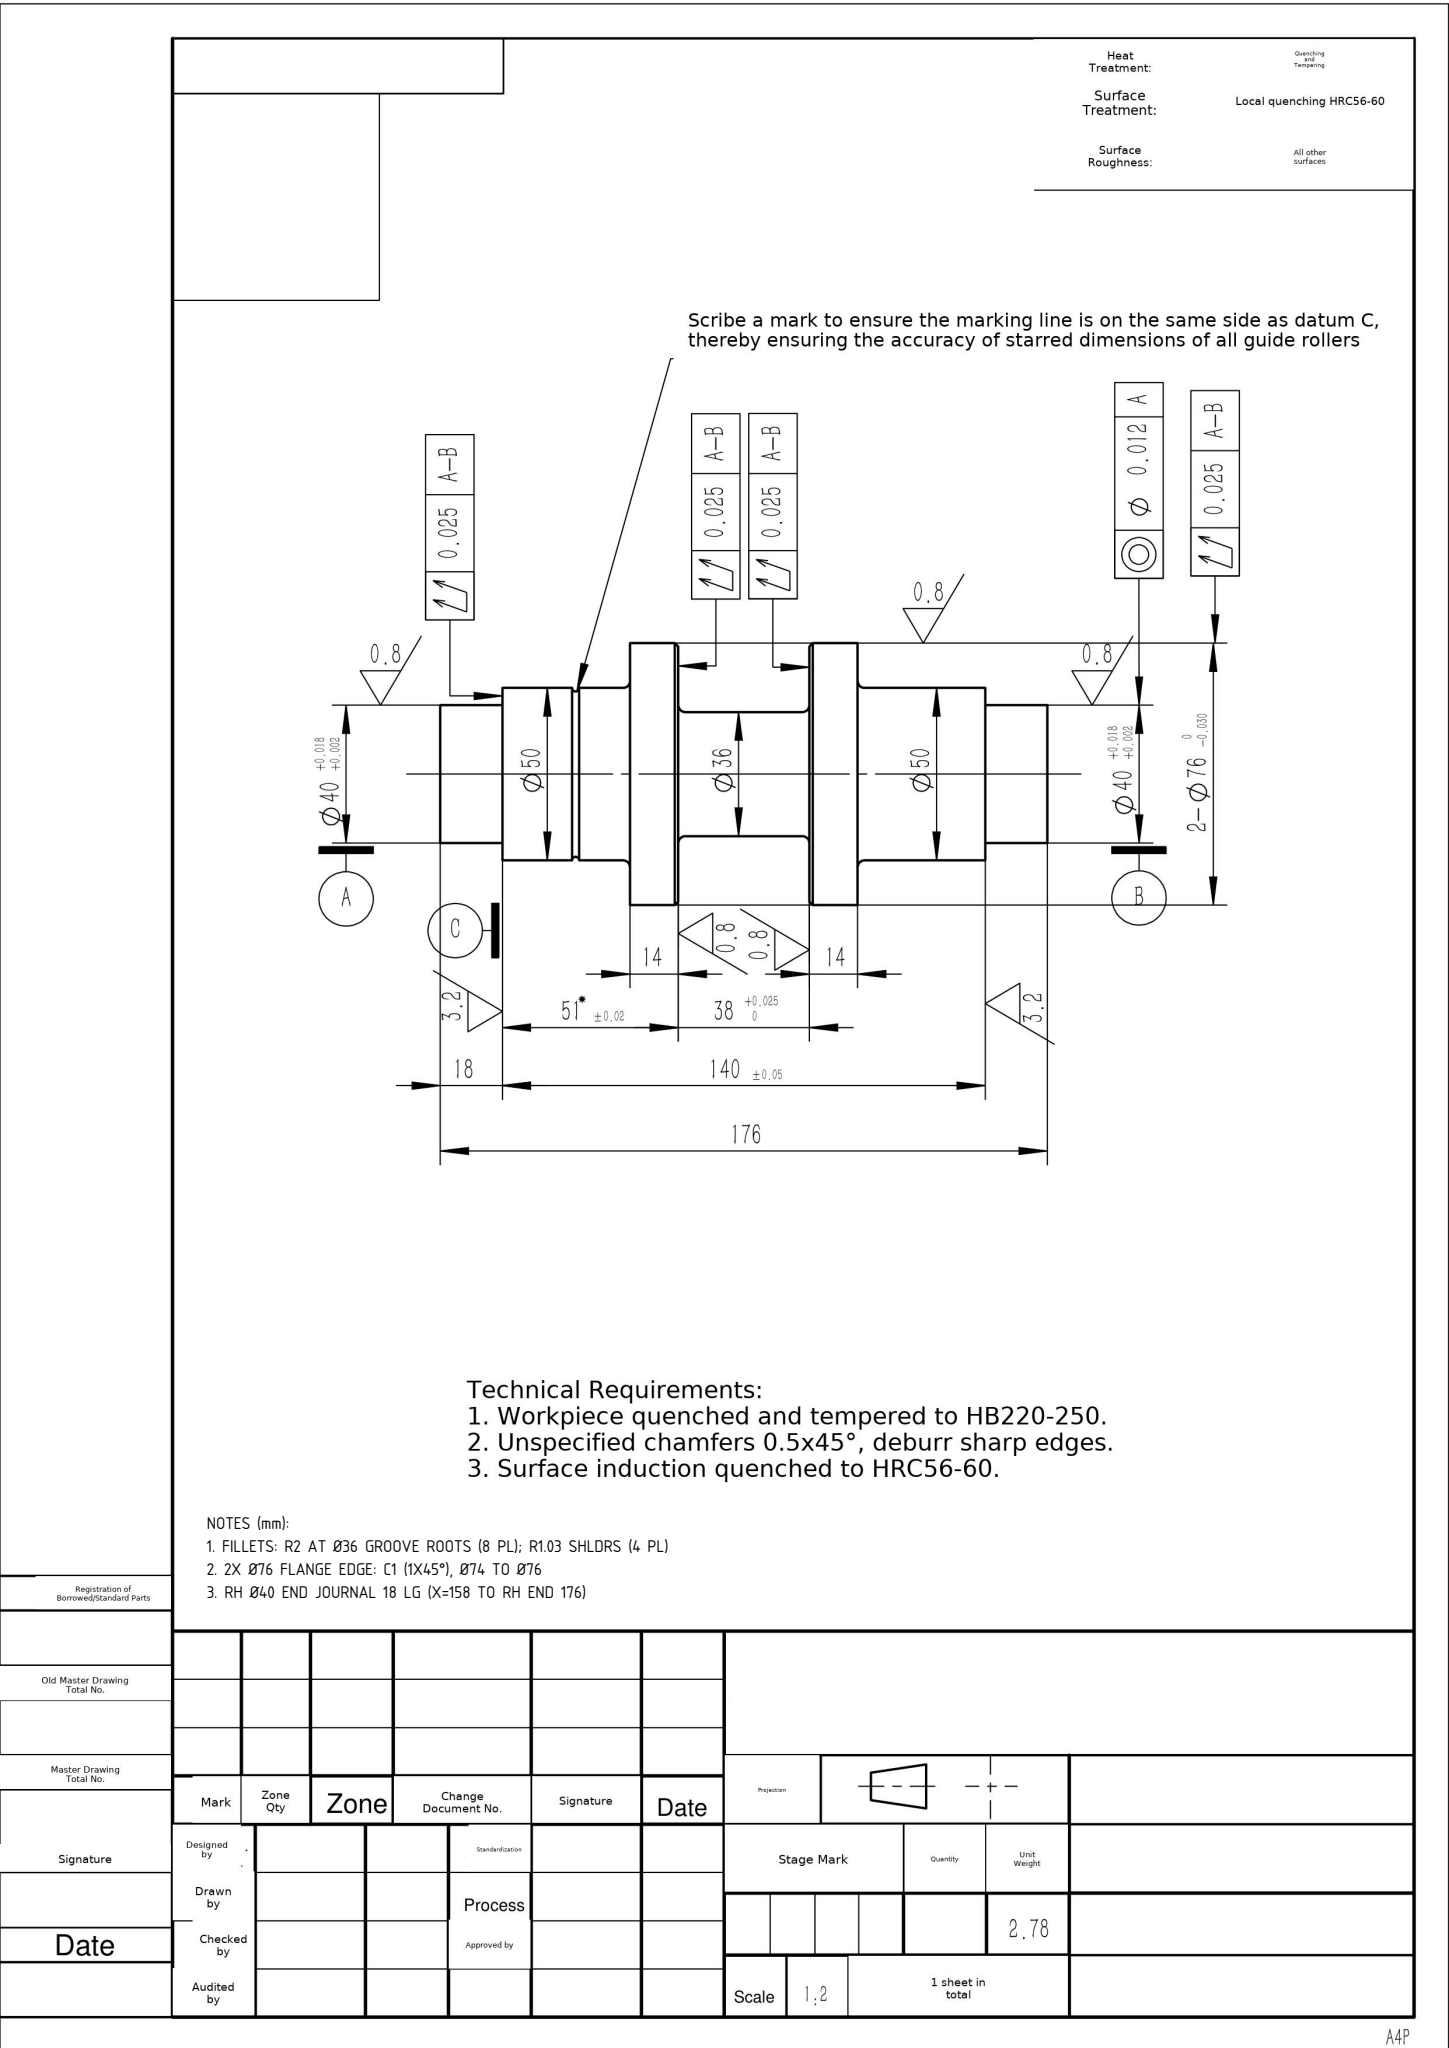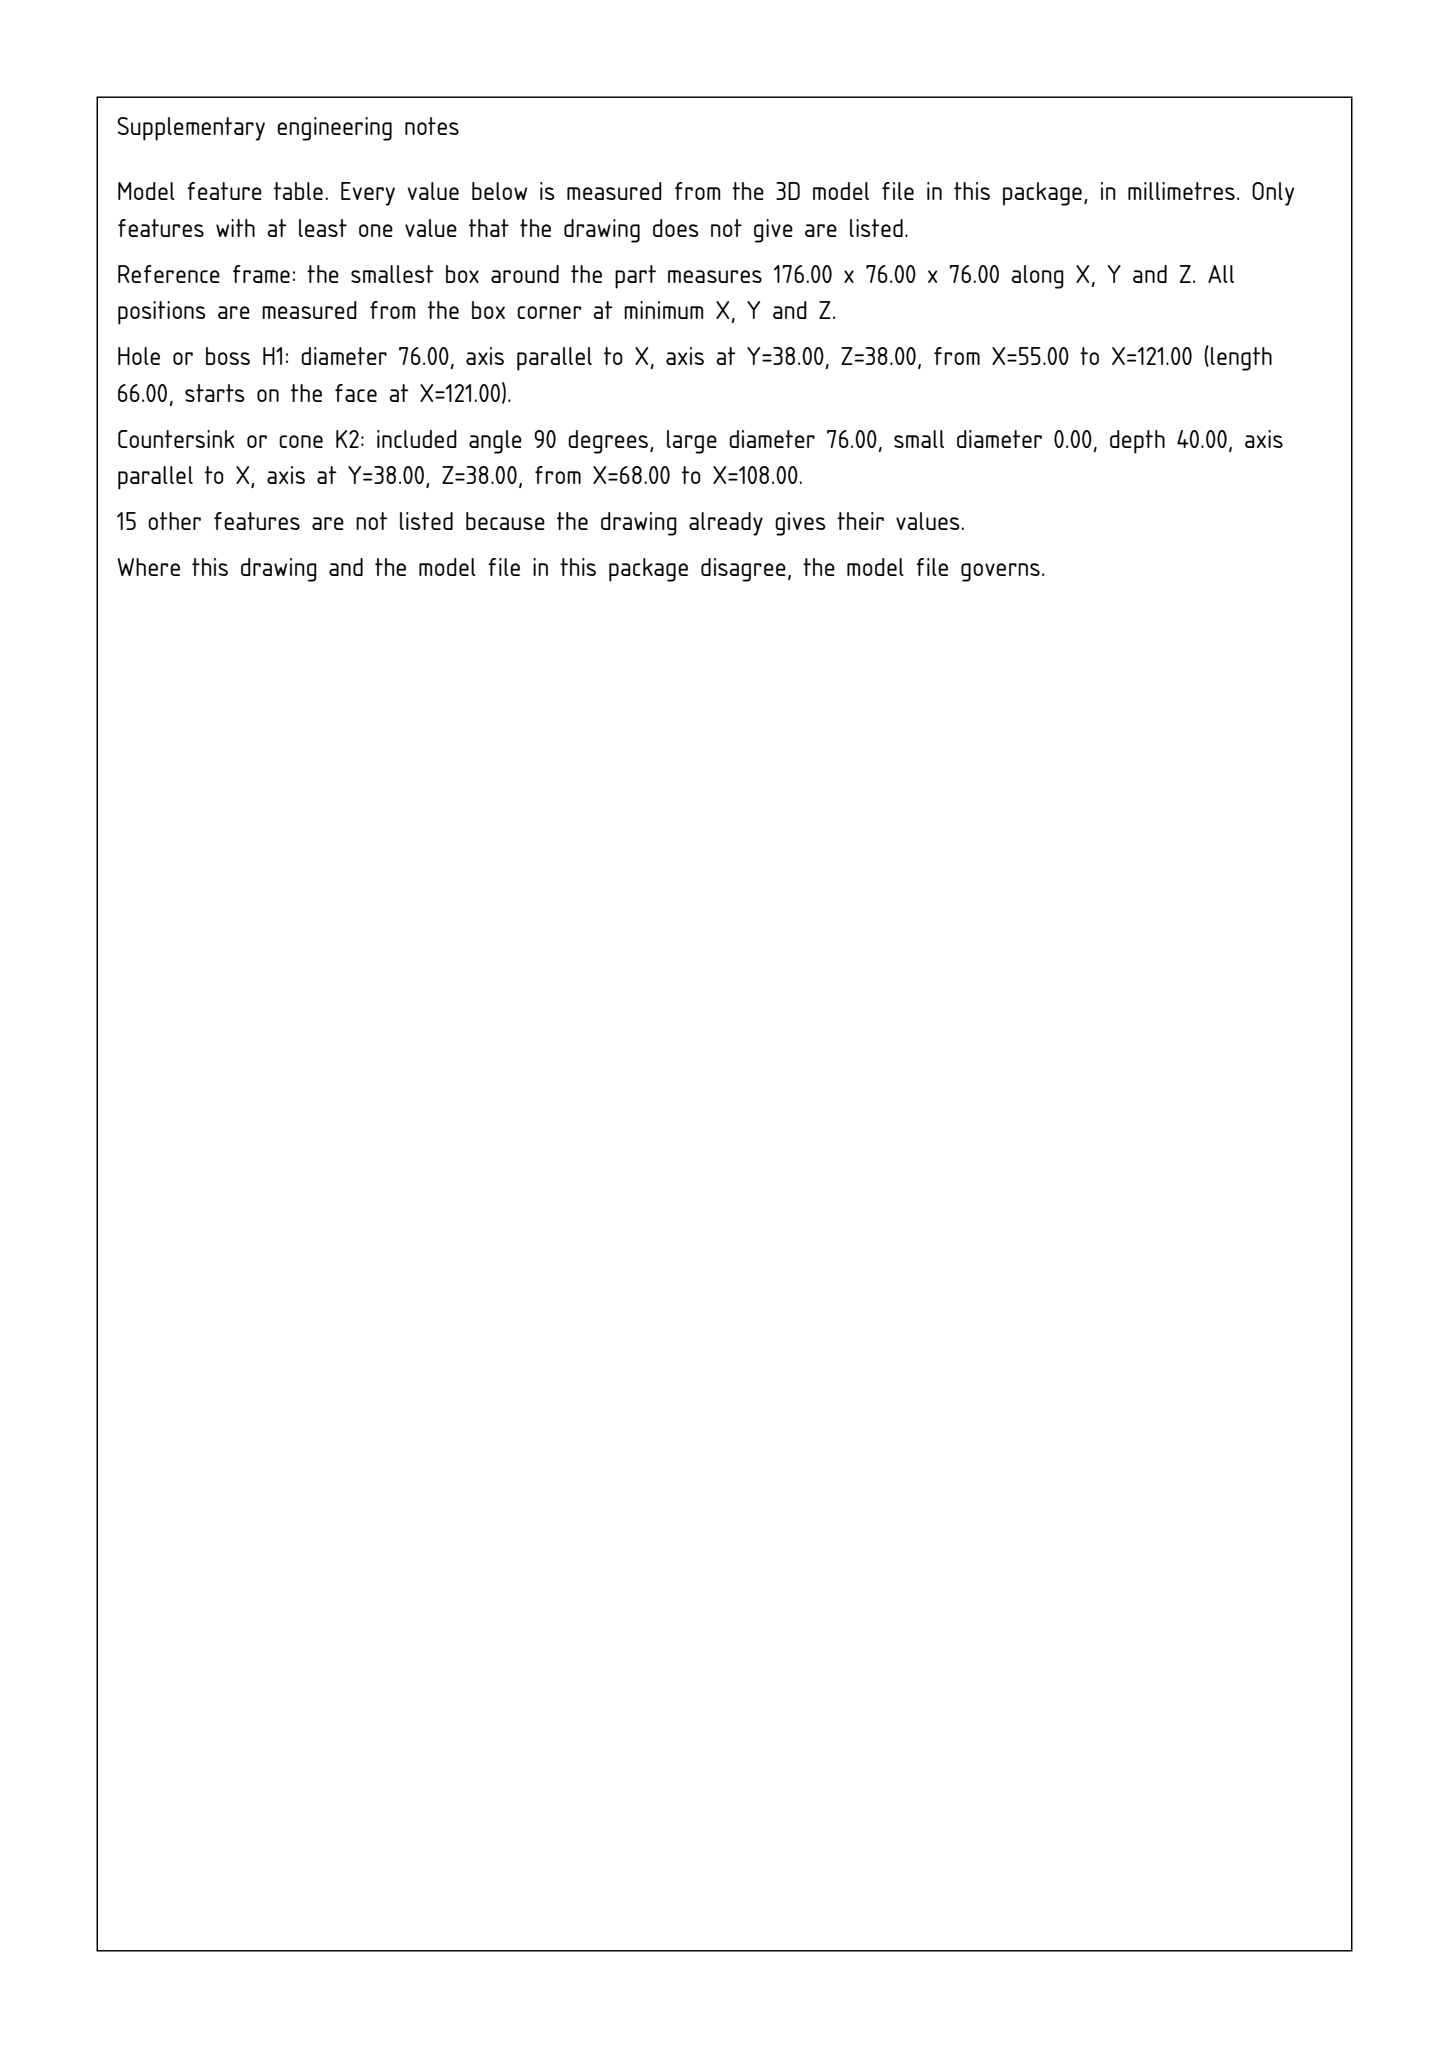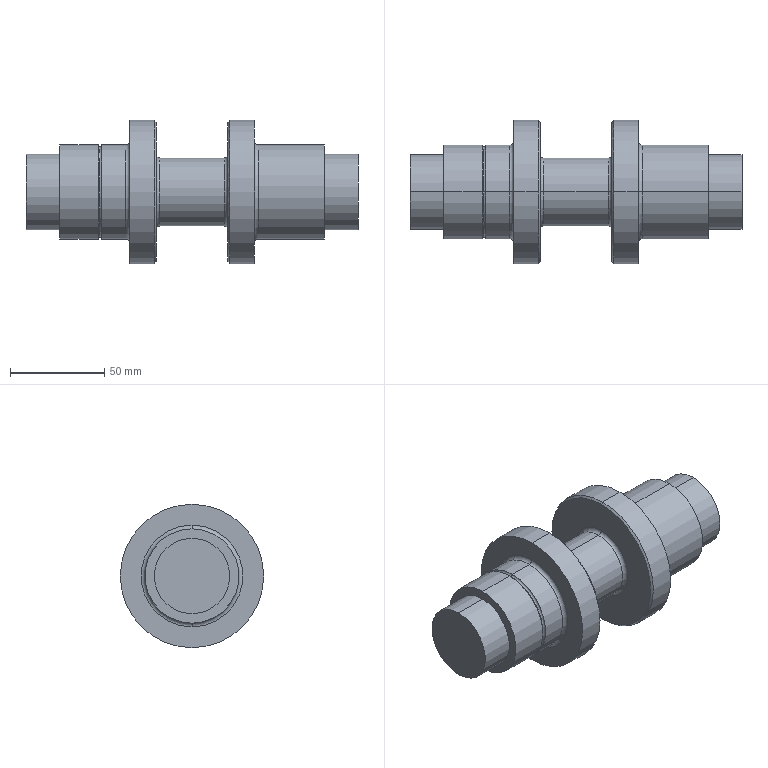Part | SolidWorks | mm | 1 solid | 40 faces | box 176 x 76 x 76 mm | volume 356219 mm3 | cylinder 16 | torus 12 | plane 8 | cone 4 | commonest cylinder face diameters 50 x6 40 x4 76 x4 36 x2
Drawing notes:
FILLETS: R2 AT Ø36 GROOVE ROOTS (8 PL); R1.03 SHLDRS (4 PL) | from the solid: fillet_radii: [2.0, 8] at Ø36 groove roots; [1.027, 4] at shoulder transitions
2X Ø76 FLANGE EDGE: C1 (1X45°), Ø74 TO Ø76 | from the solid: cones: 90° incl, ref dia 74 and 76 (2 ea) -> 1 mm x 45° bevel on Ø76 flanges
RH Ø40 END JOURNAL 18 LG (X=158 TO RH END 176) | from the solid: axis_planes x=158 and x=176; Ø40 cyl length 18
build123d program:
from build123d import *

# Parameters (mm, degrees)
SKETCH2_R           = 38
BOSS_EXTRUDE1_DEPTH = 88
SKETCH4_W           = 38
SKETCH4_H           = 20
CHAMFER1_SIZE       = 1
SKETCH5_OUTSIDE_W   = 119.244
SKETCH5_OUTSIDE_H   = 119.244
SKETCH5_OUTSIDE_R   = 20
CUT_EXTRUDE1_DEPTH  = 18
SKETCH7_OUTSIDE_W   = 119.244
SKETCH7_OUTSIDE_H   = 119.244
SKETCH7_OUTSIDE_R   = 25
CUT_EXTRUDE2_DEPTH  = 55
FILLET1_R           = 2
SKETCH8_R           = 1.027


with BuildPart() as part:
    # Sketch2 → Boss-Extrude1 (new, symmetric)
    with BuildSketch(Plane(origin=(0, 0, 0), x_dir=(0, 0, -1), z_dir=(1, 0, 0))):
        Circle(SKETCH2_R)
    extrude(amount=BOSS_EXTRUDE1_DEPTH, both=True)

    # Sketch4 → Cut-Revolve2 (revolve, cut)
    with BuildSketch(Plane(origin=(0, 0, 0), x_dir=(1, 0, 0), z_dir=(0, 1, 0)), mode=Mode.PRIVATE) as cut_revolve2_sk:
        with Locations((0, 28)):
            Rectangle(SKETCH4_W, SKETCH4_H)
    revolve(cut_revolve2_sk.sketch.rotate(Axis((0, 0, 0), (1, 0, 0)), 180), axis=Axis((0, 0, 0), (1, 0, 0)), mode=Mode.SUBTRACT)

    # Chamfer1
    chamfer1_edges = [part.edges().sort_by_distance(p)[0] for p in [
        (-19, 0, 38),
        (19, 0, 38),
    ]]
    chamfer(chamfer1_edges, length=CHAMFER1_SIZE)

    # Sketch5 outside → Cut-Extrude1 (cut)
    with BuildSketch(Plane.ZY.offset(88)):
        Rectangle(SKETCH5_OUTSIDE_W, SKETCH5_OUTSIDE_H)
        Circle(SKETCH5_OUTSIDE_R, mode=Mode.SUBTRACT)
    cut_extrude1 = extrude(amount=-CUT_EXTRUDE1_DEPTH, mode=Mode.SUBTRACT)

    # Sketch7 outside → Cut-Extrude2 (cut)
    with BuildSketch(Plane.ZY.offset(88)):
        Rectangle(SKETCH7_OUTSIDE_W, SKETCH7_OUTSIDE_H)
        Circle(SKETCH7_OUTSIDE_R, mode=Mode.SUBTRACT)
    cut_extrude2 = extrude(amount=-CUT_EXTRUDE2_DEPTH, mode=Mode.SUBTRACT)

    # Mirror1: Cut-Extrude1, Cut-Extrude2 across plane
    add(cut_extrude1.mirror(Plane(origin=(0, 0, 0), x_dir=(0, 0, 1), z_dir=(1, 0, 0))), mode=Mode.SUBTRACT)
    add(cut_extrude2.mirror(Plane(origin=(0, 0, 0), x_dir=(0, 0, 1), z_dir=(1, 0, 0))), mode=Mode.SUBTRACT)

    # Fillet1
    fillet1_edges = [part.edges().sort_by_distance(p)[0] for p in [
        (-33, 0, -25),
        (19, 0, -18),
        (-19, 0, -18),
        (33, 0, -25),
    ]]
    fillet(fillet1_edges, radius=FILLET1_R)

    # Sketch8 → Cut-Revolve4 (revolve, cut)
    with BuildSketch(Plane(origin=(0, 0, 0), x_dir=(1, 0, 0), z_dir=(0, 1, 0)), mode=Mode.PRIVATE) as cut_revolve4_sk:
        with Locations((-48.779, 25)):
            Circle(SKETCH8_R)
    revolve(cut_revolve4_sk.sketch.rotate(Axis((0, 0, 0), (-1, 0, 0)), 180), axis=Axis((0, 0, 0), (-1, 0, 0)), mode=Mode.SUBTRACT)


solid = part.part